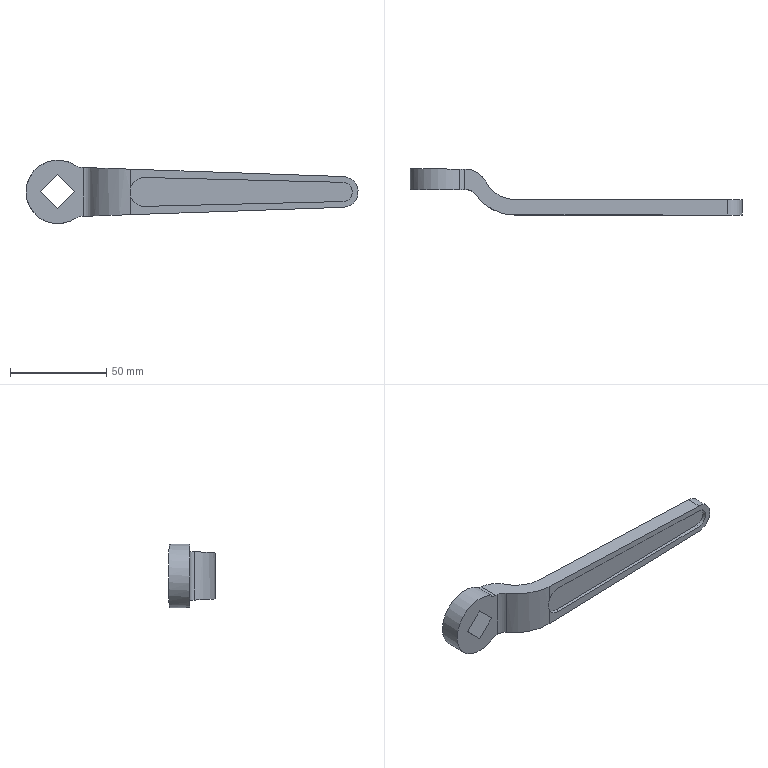Component | NX | WRENCH | 1 solid | 28 faces | volume 25957 mm3 | plane 16 | cylinder 12 | commonest cylinder face diameters 10 x5 15 x2 33 x1 16 x1 26 x1 34 x1 50 x1